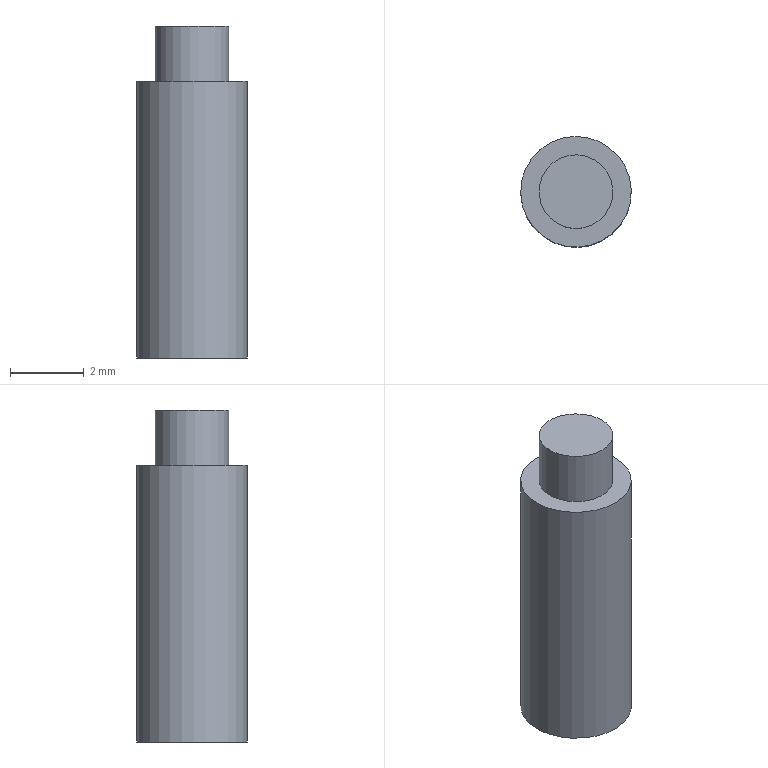Component | NX | 14__27 | 1 solid | 5 faces | box 3 x 3 x 9 mm | volume 58 mm3 | plane 3 | cylinder 2 | commonest cylinder face diameters 3 x1 2 x1
STEP:
#1=CARTESIAN_POINT('',(0.,0.,0.));
#2=DIRECTION('',(0.,0.,1.));
#3=DIRECTION('',(1.,0.,0.));
#4=AXIS2_PLACEMENT_3D('',#1,#2,#3);
#5=CARTESIAN_POINT('',(-6.352,110.209,57.932));
#6=VERTEX_POINT('',#5);
#7=CARTESIAN_POINT('',(-4.978,109.608,57.932));
#8=DIRECTION('',(0.,0.,1.));
#9=DIRECTION('',(-0.9162,0.4008,0.));
#10=AXIS2_PLACEMENT_3D('',#7,#8,#9);
#11=CIRCLE('',#10,1.5);
#12=CARTESIAN_POINT('',(-4.978,109.608,57.932));
#13=DIRECTION('',(0.,0.,1.));
#14=DIRECTION('',(-0.9162,0.4008,0.));
#15=AXIS2_PLACEMENT_3D('',#12,#13,#14);
#16=PLANE('',#15);
#17=CARTESIAN_POINT('',(0.,0.));
#18=DIRECTION('',(1.,0.));
#19=AXIS2_PLACEMENT_2D('',#17,#18);
#20=CIRCLE('',#19,1.5);
#21=(GEOMETRIC_REPRESENTATION_CONTEXT(2)PARAMETRIC_REPRESENTATION_CONTEXT()REPRESENTATION_CONTEXT('',''));
#22=DEFINITIONAL_REPRESENTATION('',(#20),#21);
#23=PCURVE('',#16,#22);
#24=CARTESIAN_POINT('',(-4.978,109.608,57.932));
#25=DIRECTION('',(0.,0.,1.));
#26=DIRECTION('',(-0.9162,0.4008,0.));
#27=AXIS2_PLACEMENT_3D('',#24,#25,#26);
#28=CYLINDRICAL_SURFACE('',#27,1.5);
#29=CARTESIAN_POINT('',(0.,0.));
#30=DIRECTION('',(1.,0.));
#31=VECTOR('',#30,1.);
#32=LINE('',#29,#31);
#33=(GEOMETRIC_REPRESENTATION_CONTEXT(2)PARAMETRIC_REPRESENTATION_CONTEXT()REPRESENTATION_CONTEXT('',''));
#34=DEFINITIONAL_REPRESENTATION('',(#32),#33);
#35=PCURVE('',#28,#34);
#36=SURFACE_CURVE('',#11,(#23,#35),.PCURVE_S1.);
#37=EDGE_CURVE('',#6,#6,#36,.T.);
#38=ORIENTED_EDGE('',*,*,#37,.F.);
#39=EDGE_LOOP('',(#38));
#40=FACE_BOUND('',#39,.T.);
#41=ADVANCED_FACE('',(#40),#16,.F.);
#42=CARTESIAN_POINT('',(-6.352,110.209,65.432));
#43=VERTEX_POINT('',#42);
#44=CARTESIAN_POINT('',(-4.978,109.608,65.432));
#45=DIRECTION('',(0.,0.,1.));
#46=DIRECTION('',(-0.9162,0.4008,0.));
#47=AXIS2_PLACEMENT_3D('',#44,#45,#46);
#48=CIRCLE('',#47,1.5);
#49=CARTESIAN_POINT('',(0.,7.5));
#50=DIRECTION('',(1.,0.));
#51=VECTOR('',#50,1.);
#52=LINE('',#49,#51);
#53=(GEOMETRIC_REPRESENTATION_CONTEXT(2)PARAMETRIC_REPRESENTATION_CONTEXT()REPRESENTATION_CONTEXT('',''));
#54=DEFINITIONAL_REPRESENTATION('',(#52),#53);
#55=PCURVE('',#28,#54);
#56=CARTESIAN_POINT('',(-5.579,108.234,65.432));
#57=DIRECTION('',(0.,0.,-1.));
#58=DIRECTION('',(0.9162,-0.4008,0.));
#59=AXIS2_PLACEMENT_3D('',#56,#57,#58);
#60=PLANE('',#59);
#61=CARTESIAN_POINT('',(-1.5,-1.5));
#62=CARTESIAN_POINT('',(-1.5,1.098));
#63=CARTESIAN_POINT('',(0.75,-0.201));
#64=CARTESIAN_POINT('',(3.,-1.5));
#65=CARTESIAN_POINT('',(0.75,-2.799));
#66=CARTESIAN_POINT('',(-1.5,-4.098));
#67=CARTESIAN_POINT('',(-1.5,-1.5));
#68=(BOUNDED_CURVE()B_SPLINE_CURVE(2,(#61,#62,#63,#64,#65,#66,#67),.UNSPECIFIED.,.T.,.F.)B_SPLINE_CURVE_WITH_KNOTS((1,2,2,2,2,1),(-2.094,0.,2.094,4.189,6.283,8.378),.UNSPECIFIED.)CURVE()GEOMETRIC_REPRESENTATION_ITEM()RATIONAL_B_SPLINE_CURVE((1.,0.5,1.,0.5,1.,0.5,1.))REPRESENTATION_ITEM(''));
#69=(GEOMETRIC_REPRESENTATION_CONTEXT(2)PARAMETRIC_REPRESENTATION_CONTEXT()REPRESENTATION_CONTEXT('',''));
#70=DEFINITIONAL_REPRESENTATION('',(#68),#69);
#71=PCURVE('',#60,#70);
#72=SURFACE_CURVE('',#48,(#55,#71),.PCURVE_S1.);
#73=EDGE_CURVE('',#43,#43,#72,.T.);
#74=ORIENTED_EDGE('',*,*,#73,.F.);
#75=CARTESIAN_POINT('',(-6.352,110.209,57.932));
#76=CARTESIAN_POINT('',(-6.352,110.209,65.432));
#77=B_SPLINE_CURVE_WITH_KNOTS('',1,(#75,#76),.UNSPECIFIED.,.F.,.F.,(2,2),(0.,7.5),.PIECEWISE_BEZIER_KNOTS.);
#78=CARTESIAN_POINT('',(0.,0.));
#79=DIRECTION('',(0.,1.));
#80=VECTOR('',#79,1.);
#81=LINE('',#78,#80);
#82=(GEOMETRIC_REPRESENTATION_CONTEXT(2)PARAMETRIC_REPRESENTATION_CONTEXT()REPRESENTATION_CONTEXT('',''));
#83=DEFINITIONAL_REPRESENTATION('',(#81),#82);
#84=PCURVE('',#28,#83);
#85=CARTESIAN_POINT('',(6.283,0.));
#86=DIRECTION('',(0.,1.));
#87=VECTOR('',#86,1.);
#88=LINE('',#85,#87);
#89=(GEOMETRIC_REPRESENTATION_CONTEXT(2)PARAMETRIC_REPRESENTATION_CONTEXT()REPRESENTATION_CONTEXT('',''));
#90=DEFINITIONAL_REPRESENTATION('',(#88),#89);
#91=PCURVE('',#28,#90);
#92=SEAM_CURVE('',#77,(#84,#91),.PCURVE_S1.);
#93=EDGE_CURVE('',#6,#43,#92,.T.);
#94=ORIENTED_EDGE('',*,*,#93,.F.);
#95=ORIENTED_EDGE('',*,*,#37,.T.);
#96=ORIENTED_EDGE('',*,*,#93,.T.);
#97=EDGE_LOOP('',(#74,#94,#95,#96));
#98=FACE_BOUND('',#97,.T.);
#99=ADVANCED_FACE('',(#98),#28,.T.);
#100=CARTESIAN_POINT('',(-5.894,110.009,65.432));
#101=VERTEX_POINT('',#100);
#102=CARTESIAN_POINT('',(-4.978,109.608,65.432));
#103=DIRECTION('',(0.,0.,1.));
#104=DIRECTION('',(-0.9162,0.4008,0.));
#105=AXIS2_PLACEMENT_3D('',#102,#103,#104);
#106=CIRCLE('',#105,1.);
#107=CARTESIAN_POINT('',(-1.,-1.5));
#108=CARTESIAN_POINT('',(-1.,0.2321));
#109=CARTESIAN_POINT('',(0.5,-0.634));
#110=CARTESIAN_POINT('',(2.,-1.5));
#111=CARTESIAN_POINT('',(0.5,-2.366));
#112=CARTESIAN_POINT('',(-1.,-3.232));
#113=CARTESIAN_POINT('',(-1.,-1.5));
#114=(BOUNDED_CURVE()B_SPLINE_CURVE(2,(#107,#108,#109,#110,#111,#112,#113),.UNSPECIFIED.,.T.,.F.)B_SPLINE_CURVE_WITH_KNOTS((1,2,2,2,2,1),(-2.094,0.,2.094,4.189,6.283,8.378),.UNSPECIFIED.)CURVE()GEOMETRIC_REPRESENTATION_ITEM()RATIONAL_B_SPLINE_CURVE((1.,0.5,1.,0.5,1.,0.5,1.))REPRESENTATION_ITEM(''));
#115=(GEOMETRIC_REPRESENTATION_CONTEXT(2)PARAMETRIC_REPRESENTATION_CONTEXT()REPRESENTATION_CONTEXT('',''));
#116=DEFINITIONAL_REPRESENTATION('',(#114),#115);
#117=PCURVE('',#60,#116);
#118=CARTESIAN_POINT('',(-4.978,109.608,57.932));
#119=DIRECTION('',(0.,0.,1.));
#120=DIRECTION('',(-0.9162,0.4008,0.));
#121=AXIS2_PLACEMENT_3D('',#118,#119,#120);
#122=CYLINDRICAL_SURFACE('',#121,1.);
#123=CARTESIAN_POINT('',(0.,7.5));
#124=DIRECTION('',(1.,0.));
#125=VECTOR('',#124,1.);
#126=LINE('',#123,#125);
#127=(GEOMETRIC_REPRESENTATION_CONTEXT(2)PARAMETRIC_REPRESENTATION_CONTEXT()REPRESENTATION_CONTEXT('',''));
#128=DEFINITIONAL_REPRESENTATION('',(#126),#127);
#129=PCURVE('',#122,#128);
#130=SURFACE_CURVE('',#106,(#117,#129),.PCURVE_S1.);
#131=EDGE_CURVE('',#101,#101,#130,.T.);
#132=ORIENTED_EDGE('',*,*,#131,.F.);
#133=EDGE_LOOP('',(#132));
#134=FACE_BOUND('',#133,.T.);
#135=ORIENTED_EDGE('',*,*,#73,.T.);
#136=EDGE_LOOP('',(#135));
#137=FACE_BOUND('',#136,.T.);
#138=ADVANCED_FACE('',(#134,#137),#60,.F.);
#139=CARTESIAN_POINT('',(-5.894,110.009,66.932));
#140=VERTEX_POINT('',#139);
#141=CARTESIAN_POINT('',(-4.978,109.608,66.932));
#142=DIRECTION('',(0.,0.,1.));
#143=DIRECTION('',(-0.9162,0.4008,0.));
#144=AXIS2_PLACEMENT_3D('',#141,#142,#143);
#145=CIRCLE('',#144,1.);
#146=CARTESIAN_POINT('',(0.,9.));
#147=DIRECTION('',(1.,0.));
#148=VECTOR('',#147,1.);
#149=LINE('',#146,#148);
#150=(GEOMETRIC_REPRESENTATION_CONTEXT(2)PARAMETRIC_REPRESENTATION_CONTEXT()REPRESENTATION_CONTEXT('',''));
#151=DEFINITIONAL_REPRESENTATION('',(#149),#150);
#152=PCURVE('',#122,#151);
#153=CARTESIAN_POINT('',(-5.379,108.692,66.932));
#154=DIRECTION('',(0.,0.,-1.));
#155=DIRECTION('',(0.9162,-0.4008,0.));
#156=AXIS2_PLACEMENT_3D('',#153,#154,#155);
#157=PLANE('',#156);
#158=CARTESIAN_POINT('',(-1.,-1.));
#159=CARTESIAN_POINT('',(-1.,0.7321));
#160=CARTESIAN_POINT('',(0.5,-0.134));
#161=CARTESIAN_POINT('',(2.,-1.));
#162=CARTESIAN_POINT('',(0.5,-1.866));
#163=CARTESIAN_POINT('',(-1.,-2.732));
#164=CARTESIAN_POINT('',(-1.,-1.));
#165=(BOUNDED_CURVE()B_SPLINE_CURVE(2,(#158,#159,#160,#161,#162,#163,#164),.UNSPECIFIED.,.T.,.F.)B_SPLINE_CURVE_WITH_KNOTS((1,2,2,2,2,1),(-2.094,0.,2.094,4.189,6.283,8.378),.UNSPECIFIED.)CURVE()GEOMETRIC_REPRESENTATION_ITEM()RATIONAL_B_SPLINE_CURVE((1.,0.5,1.,0.5,1.,0.5,1.))REPRESENTATION_ITEM(''));
#166=(GEOMETRIC_REPRESENTATION_CONTEXT(2)PARAMETRIC_REPRESENTATION_CONTEXT()REPRESENTATION_CONTEXT('',''));
#167=DEFINITIONAL_REPRESENTATION('',(#165),#166);
#168=PCURVE('',#157,#167);
#169=SURFACE_CURVE('',#145,(#152,#168),.PCURVE_S1.);
#170=EDGE_CURVE('',#140,#140,#169,.T.);
#171=ORIENTED_EDGE('',*,*,#170,.F.);
#172=CARTESIAN_POINT('',(-5.894,110.009,65.432));
#173=CARTESIAN_POINT('',(-5.894,110.009,66.932));
#174=B_SPLINE_CURVE_WITH_KNOTS('',1,(#172,#173),.UNSPECIFIED.,.F.,.F.,(2,2),(7.5,9.),.PIECEWISE_BEZIER_KNOTS.);
#175=CARTESIAN_POINT('',(0.,0.));
#176=DIRECTION('',(0.,1.));
#177=VECTOR('',#176,1.);
#178=LINE('',#175,#177);
#179=(GEOMETRIC_REPRESENTATION_CONTEXT(2)PARAMETRIC_REPRESENTATION_CONTEXT()REPRESENTATION_CONTEXT('',''));
#180=DEFINITIONAL_REPRESENTATION('',(#178),#179);
#181=PCURVE('',#122,#180);
#182=CARTESIAN_POINT('',(6.283,0.));
#183=DIRECTION('',(0.,1.));
#184=VECTOR('',#183,1.);
#185=LINE('',#182,#184);
#186=(GEOMETRIC_REPRESENTATION_CONTEXT(2)PARAMETRIC_REPRESENTATION_CONTEXT()REPRESENTATION_CONTEXT('',''));
#187=DEFINITIONAL_REPRESENTATION('',(#185),#186);
#188=PCURVE('',#122,#187);
#189=SEAM_CURVE('',#174,(#181,#188),.PCURVE_S1.);
#190=EDGE_CURVE('',#101,#140,#189,.T.);
#191=ORIENTED_EDGE('',*,*,#190,.F.);
#192=ORIENTED_EDGE('',*,*,#131,.T.);
#193=ORIENTED_EDGE('',*,*,#190,.T.);
#194=EDGE_LOOP('',(#171,#191,#192,#193));
#195=FACE_BOUND('',#194,.T.);
#196=ADVANCED_FACE('',(#195),#122,.T.);
#197=ORIENTED_EDGE('',*,*,#170,.T.);
#198=EDGE_LOOP('',(#197));
#199=FACE_BOUND('',#198,.T.);
#200=ADVANCED_FACE('',(#199),#157,.F.);
#201=CLOSED_SHELL('',(#41,#99,#138,#196,#200));
#202=MANIFOLD_SOLID_BREP('',#201);
#203=(LENGTH_UNIT()NAMED_UNIT(*)SI_UNIT(.MILLI.,.METRE.));
#204=UNCERTAINTY_MEASURE_WITH_UNIT(LENGTH_MEASURE(0.00001),#203,'','');
#205=(NAMED_UNIT(*)PLANE_ANGLE_UNIT()SI_UNIT($,.RADIAN.));
#206=(NAMED_UNIT(*)SI_UNIT($,.STERADIAN.)SOLID_ANGLE_UNIT());
#207=(GEOMETRIC_REPRESENTATION_CONTEXT(3)GLOBAL_UNCERTAINTY_ASSIGNED_CONTEXT((#204))GLOBAL_UNIT_ASSIGNED_CONTEXT((#203,#205,#206))REPRESENTATION_CONTEXT('',''));
#208=ADVANCED_BREP_SHAPE_REPRESENTATION('',(#4,#202),#207);